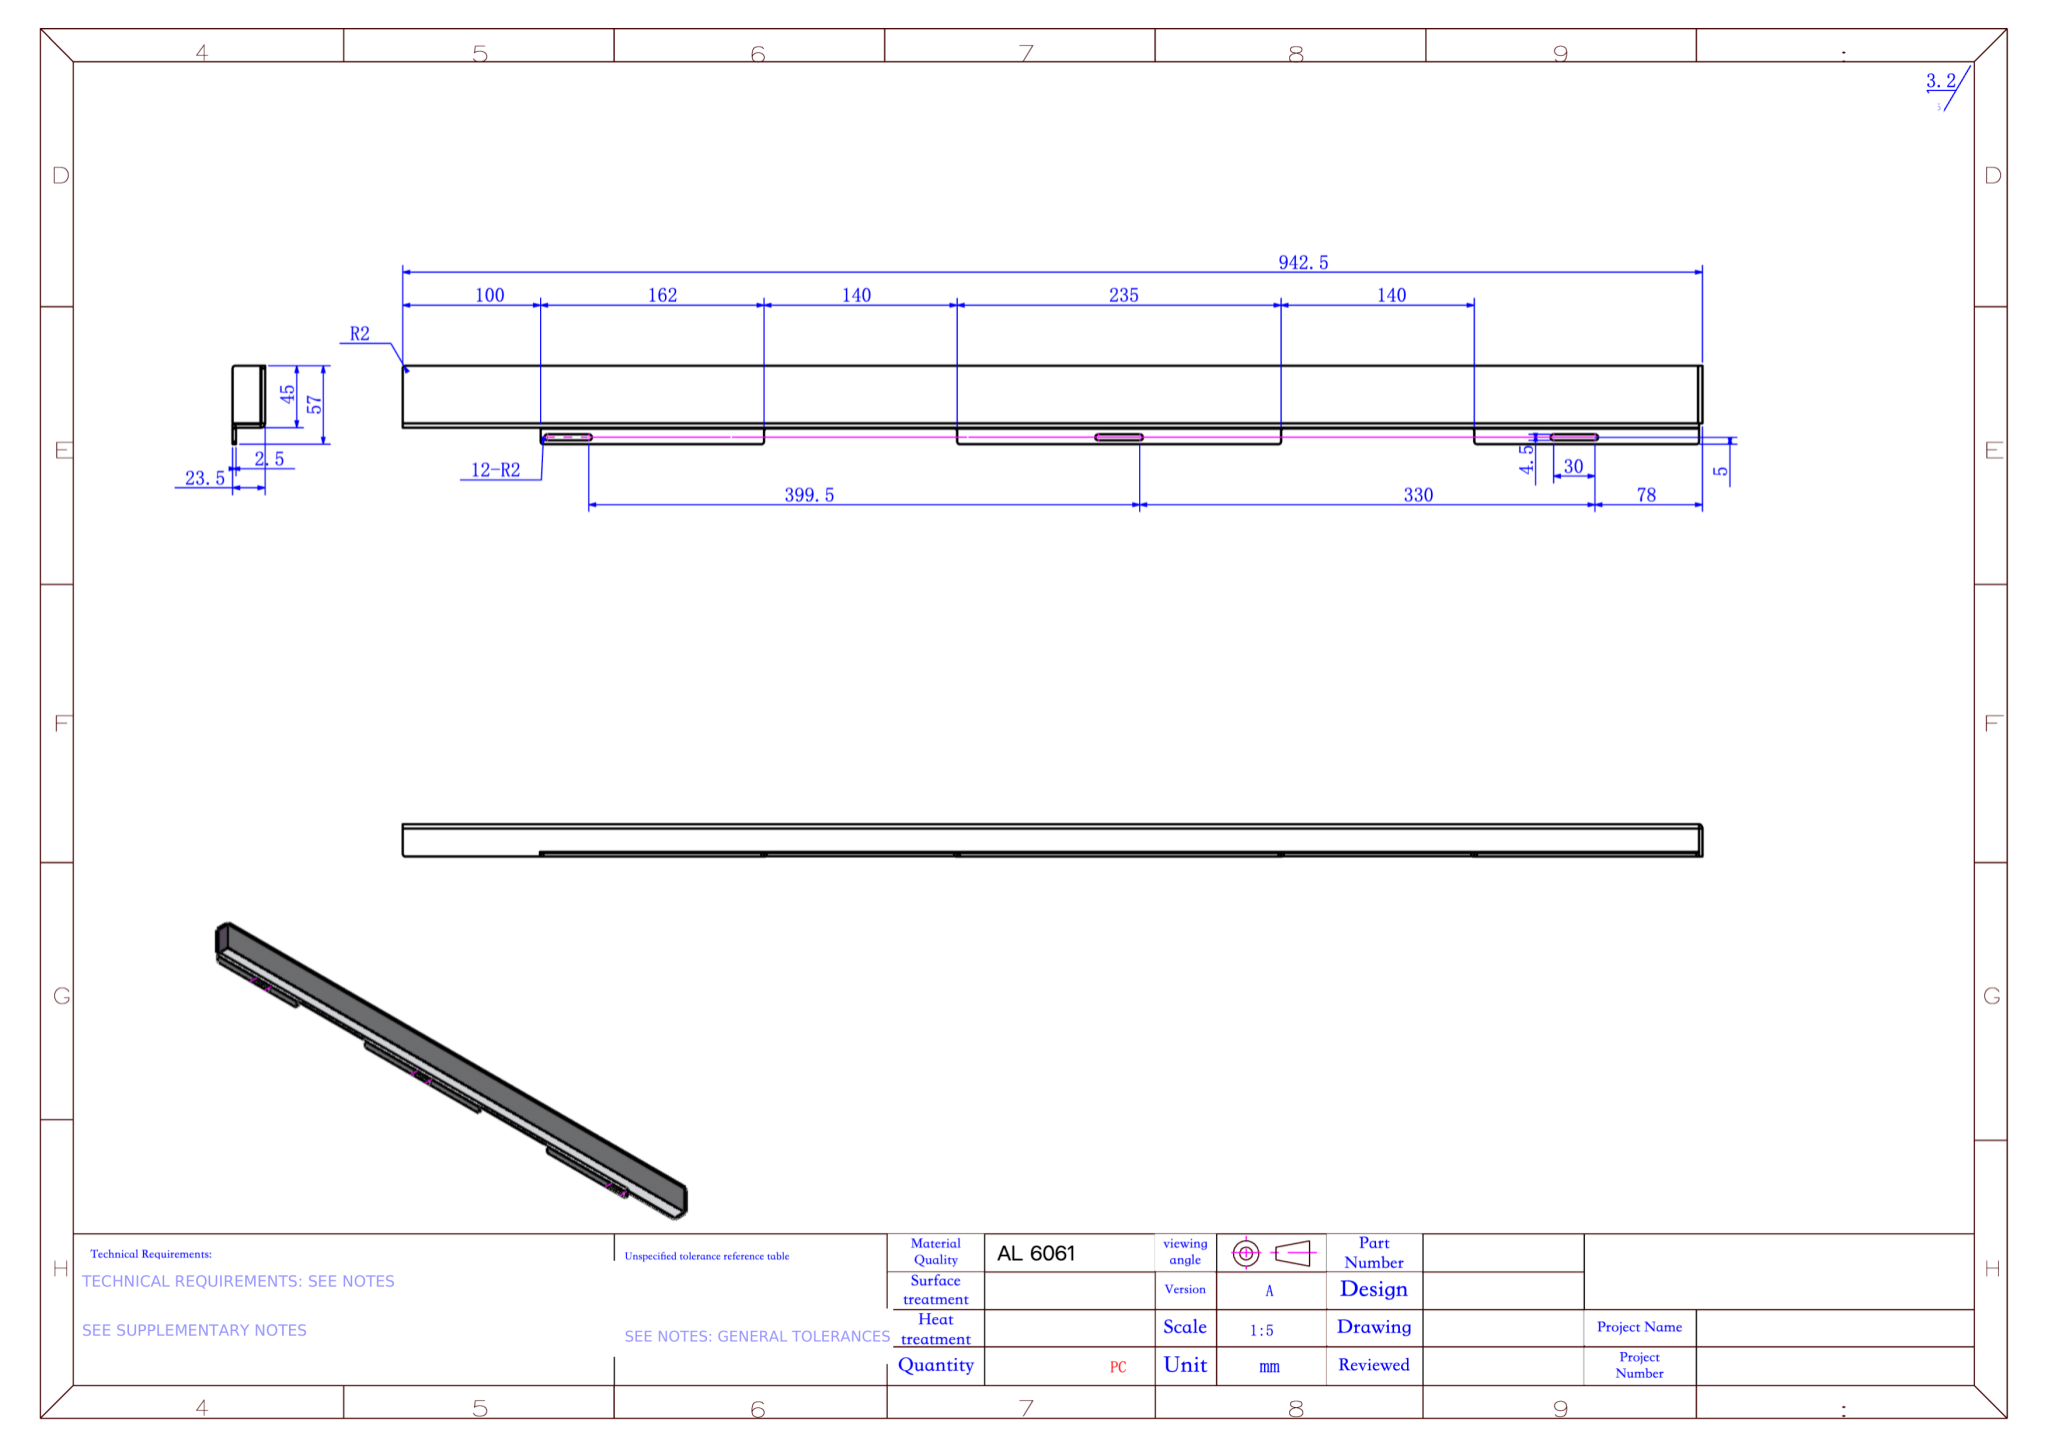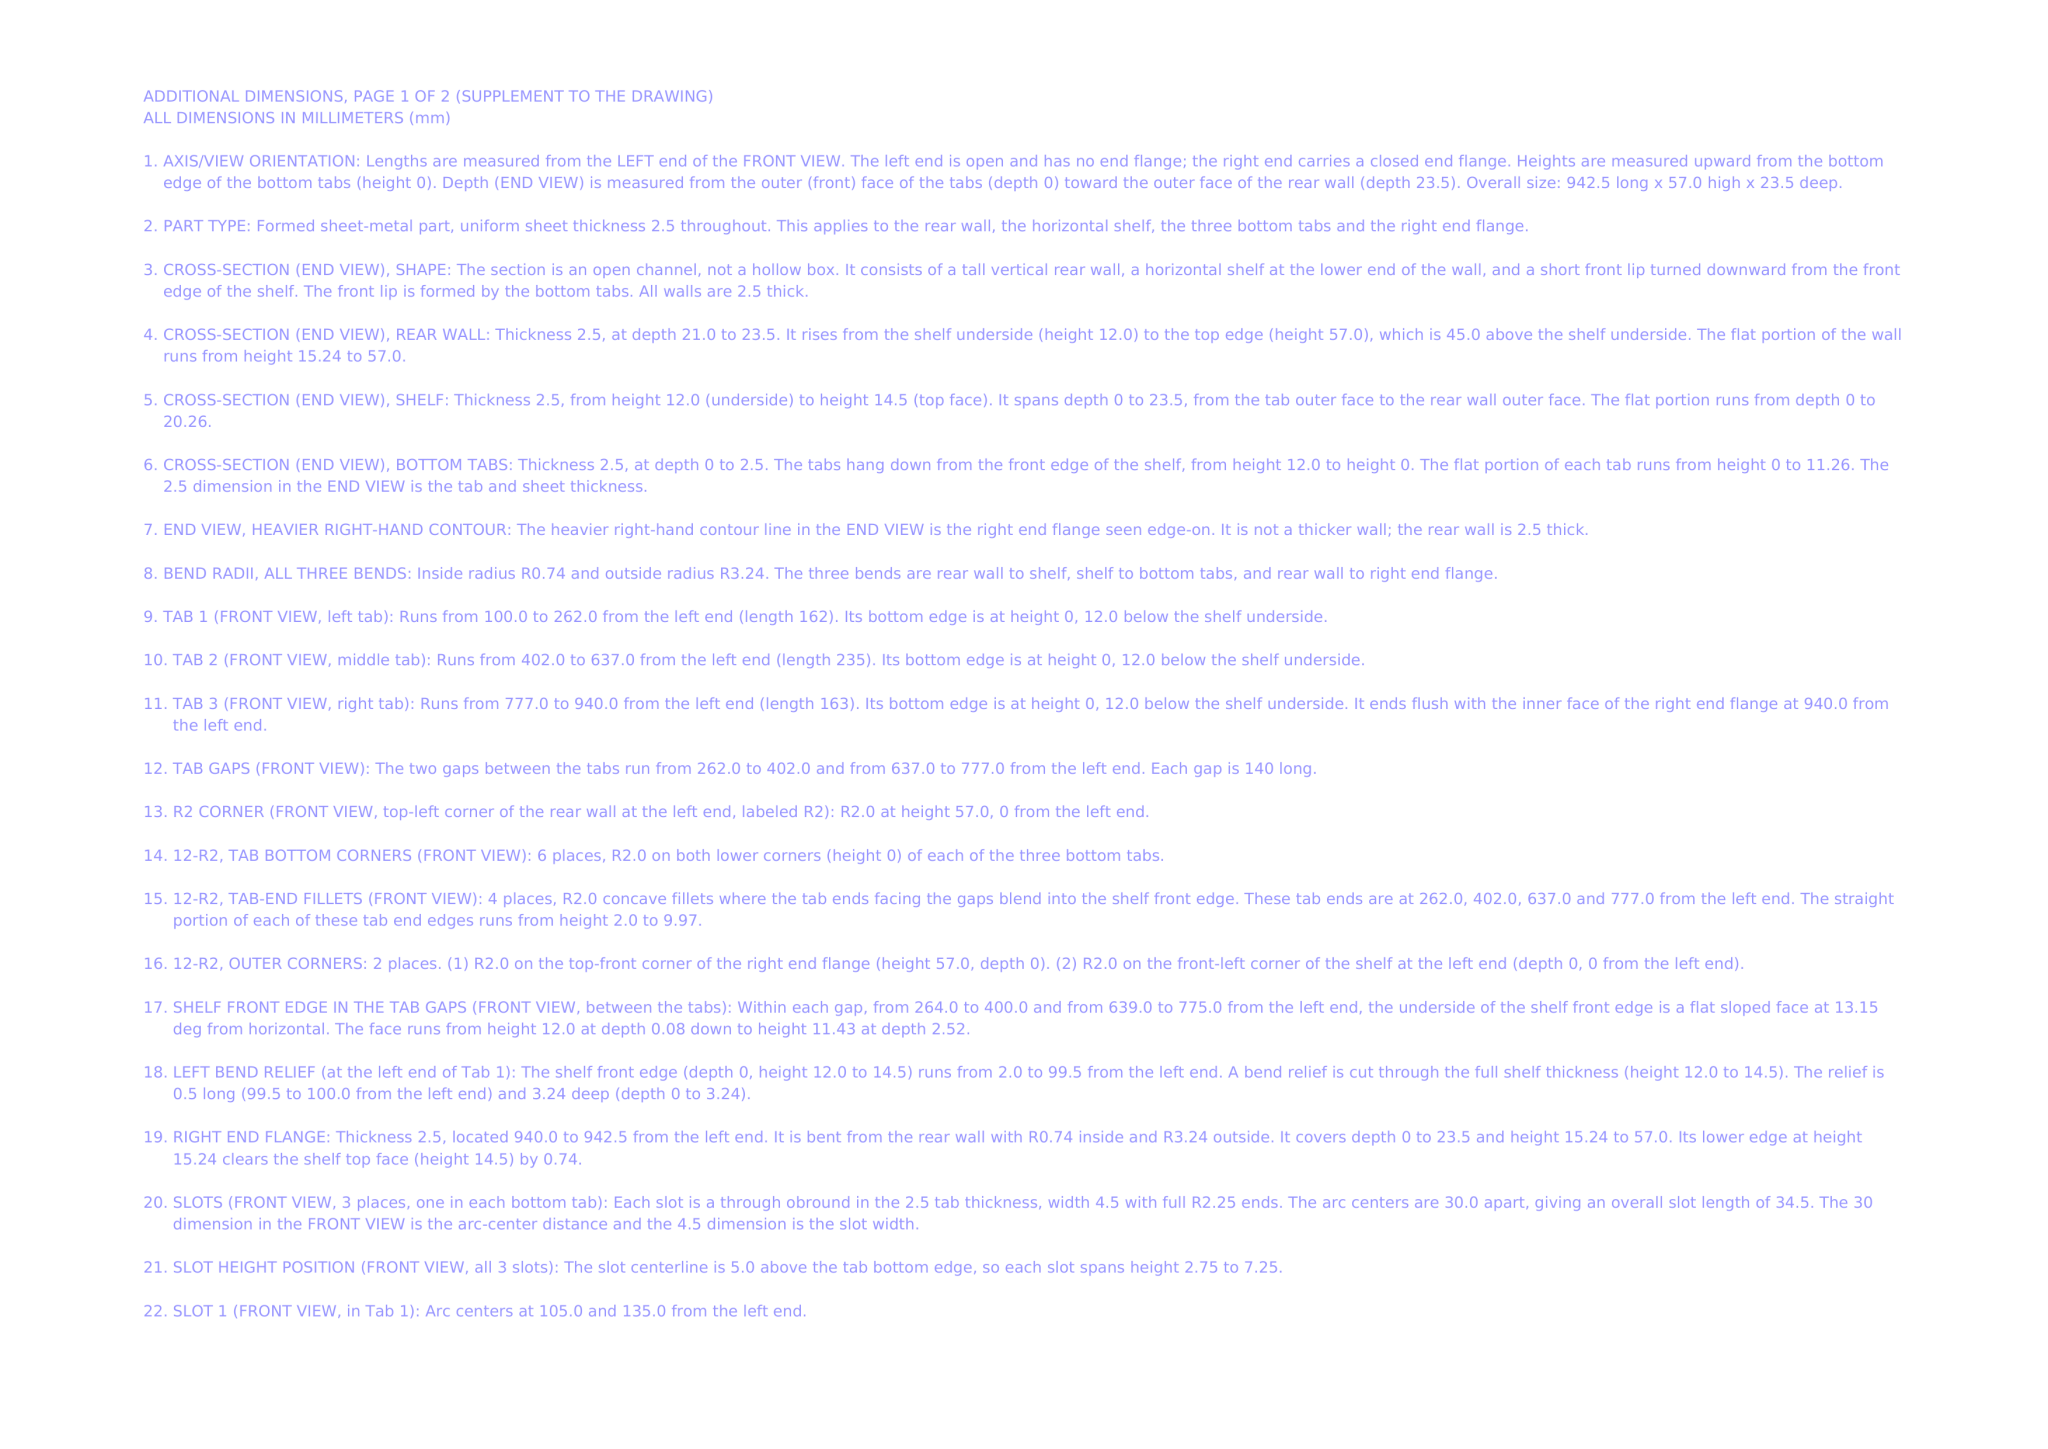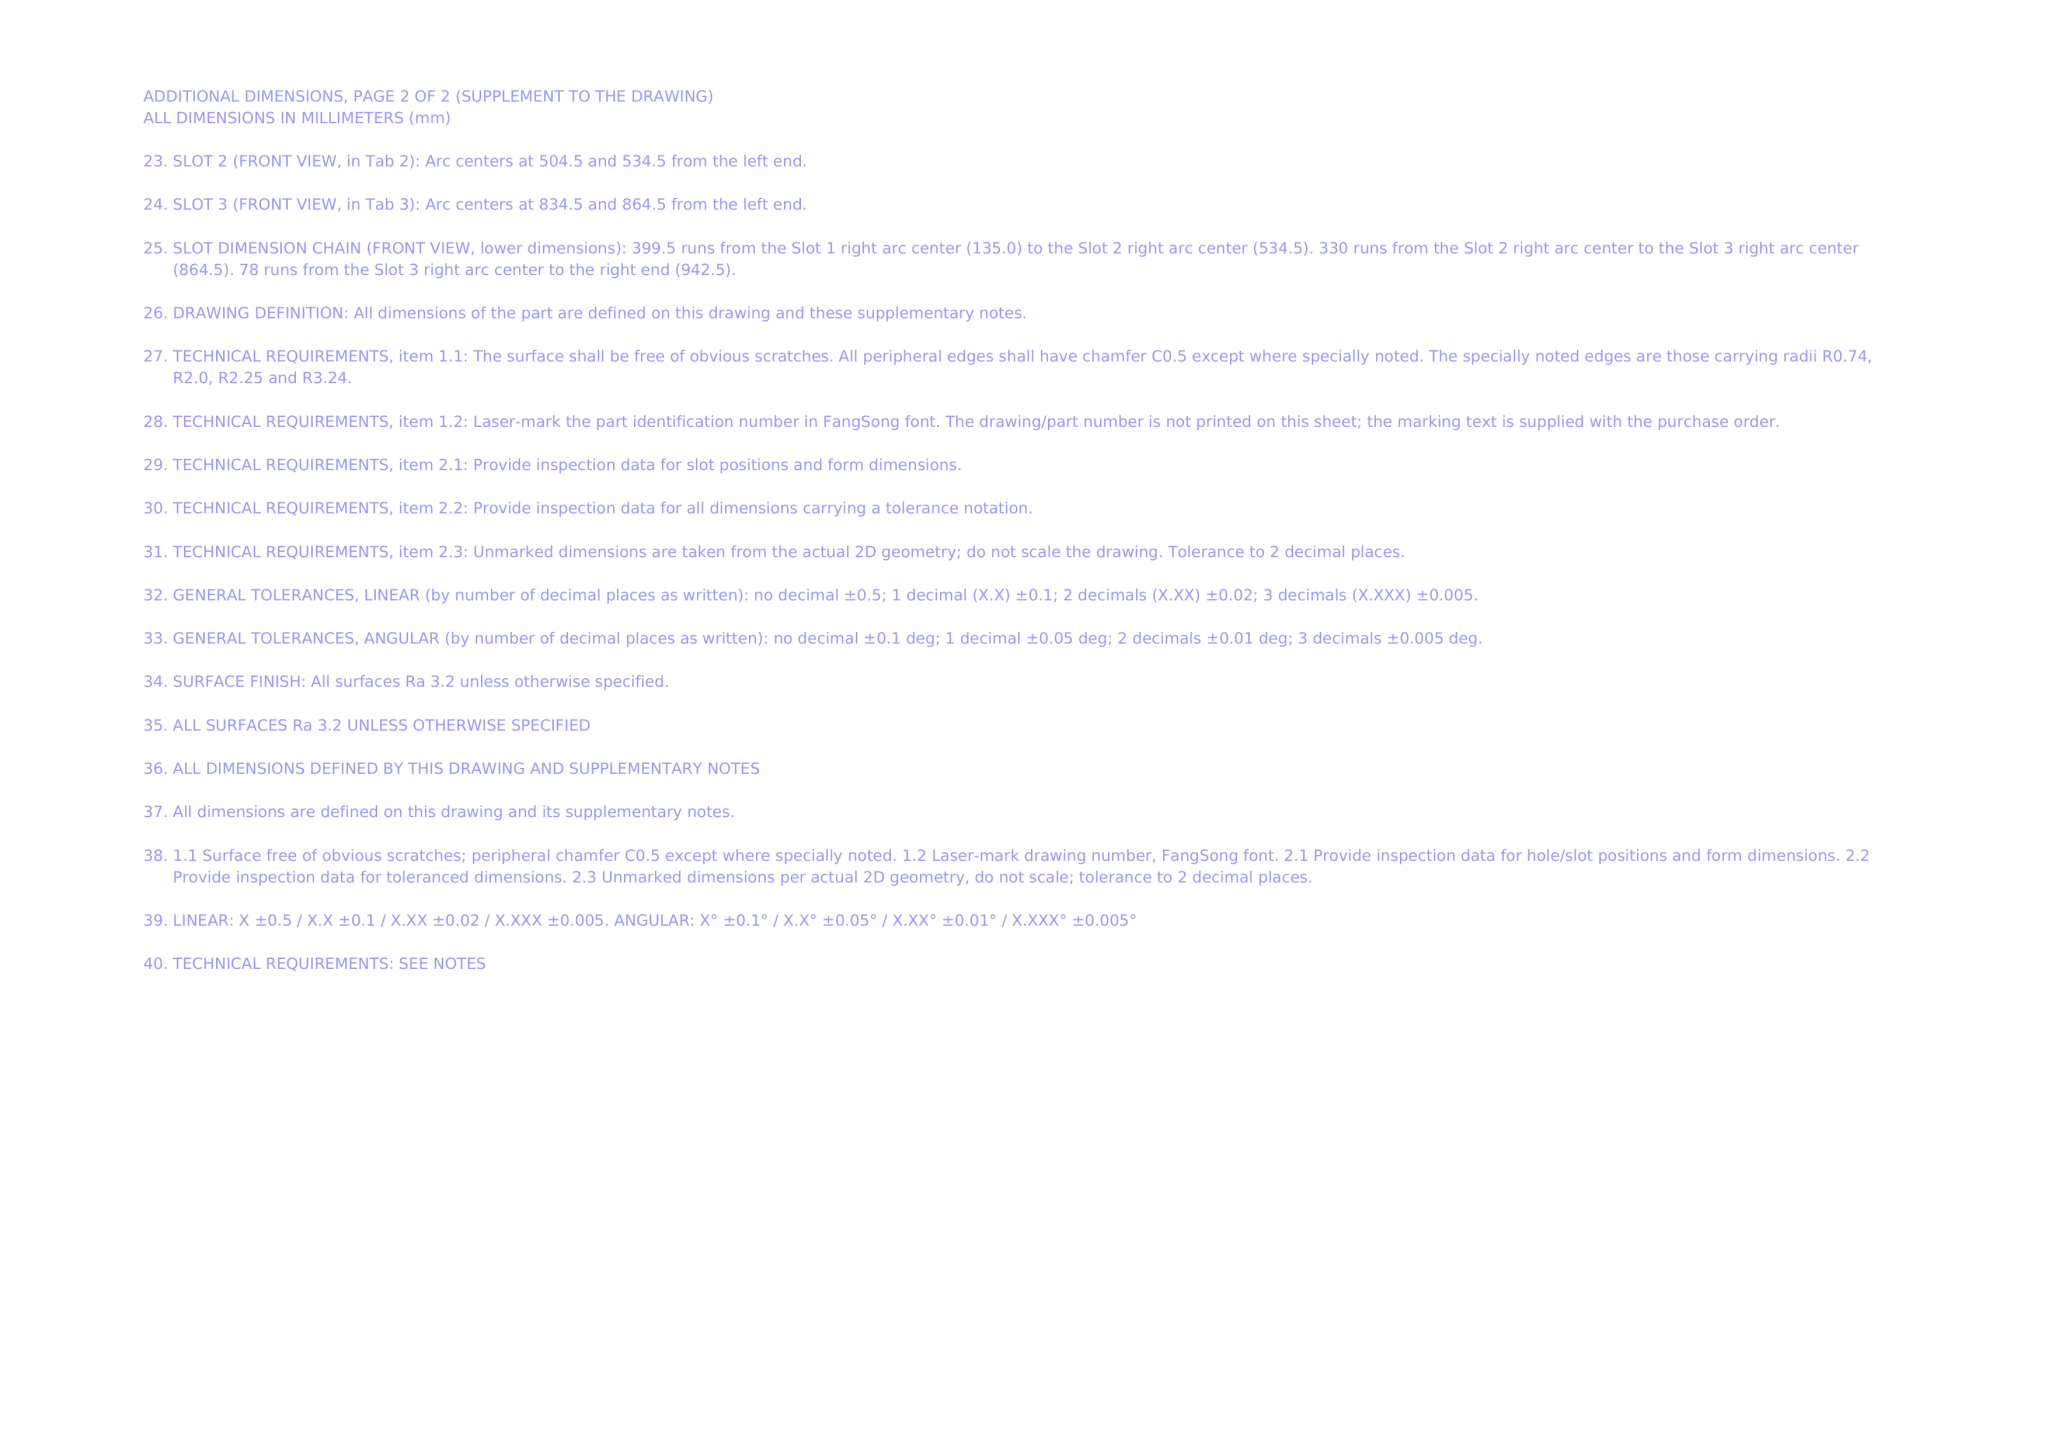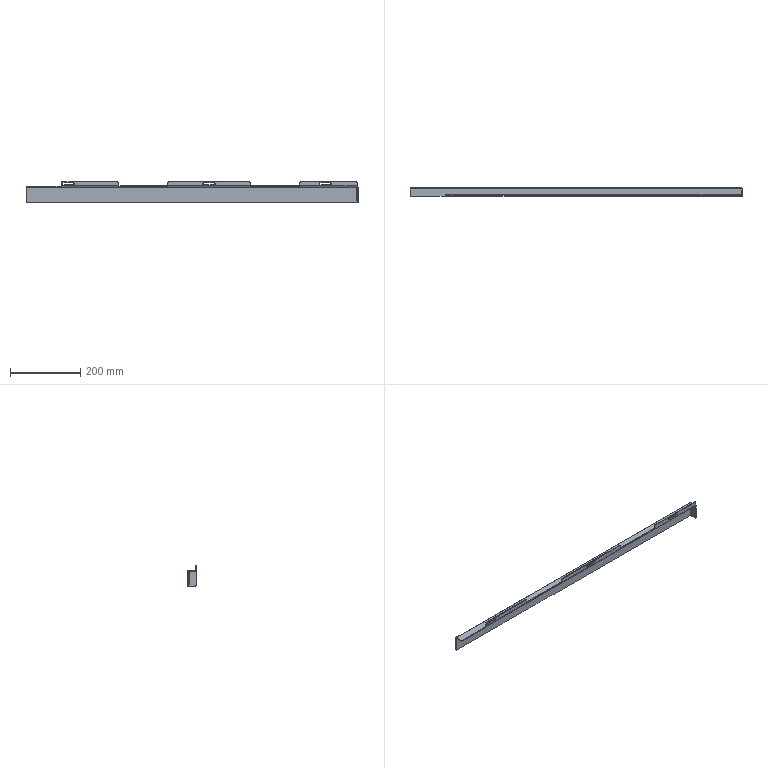Part | NX | mm | 1 solid | 71 faces | box 942.5 x 23.5 x 57 mm | volume 169520 mm3 | plane 46 | cylinder 25 | commonest cylinder face diameters 4 x13 4.5 x6 1.473 x3 6.473 x3